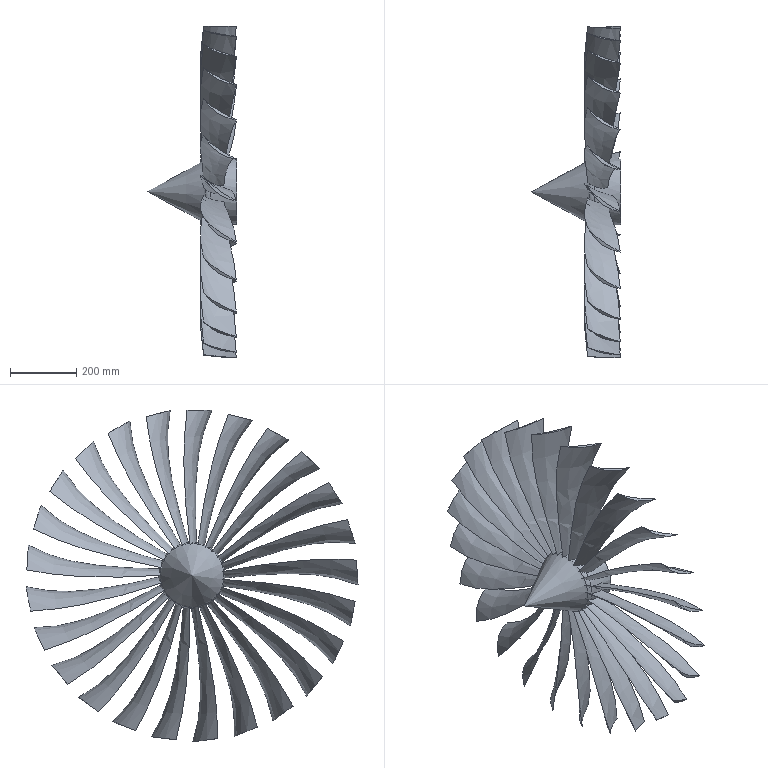Component | NX | TURBOFAN_ENGINE | 1 solid | 109 faces | volume 8834727 mm3 | spline 50 | plane 30 | torus 25 | cylinder 3 | cone 1 | commonest cylinder face diameters 200 x2 80 x1